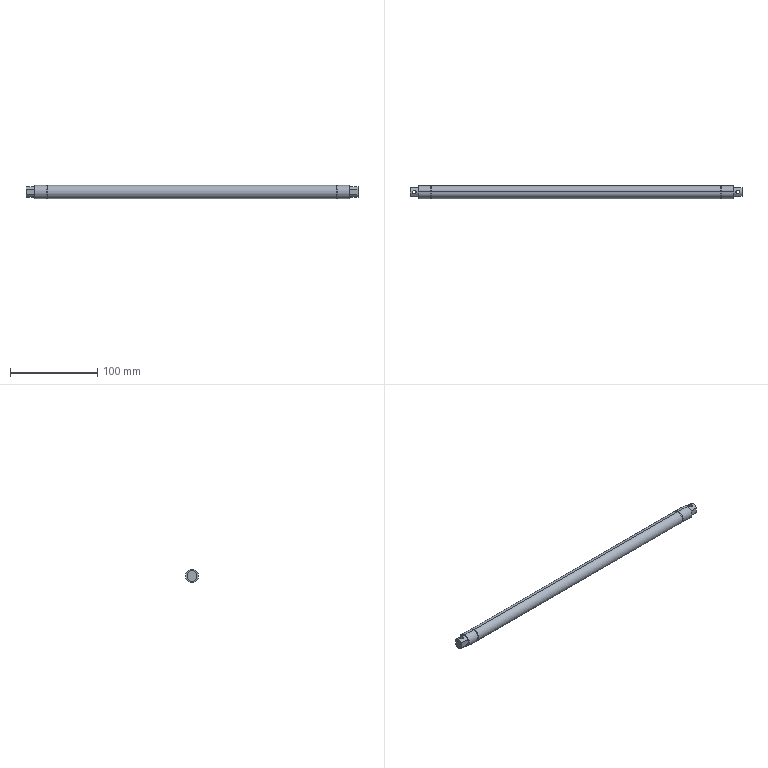Component | SolidWorks | 01-12MarkingMachinePrintingRollerAxis-1 | 1 solid | 32 faces | box 380 x 15 x 15 mm | volume 65336 mm3 | cylinder 20 | plane 12 | commonest cylinder face diameters 15 x6 12 x6 4.2 x4 14.3 x4 | material A3 Steel
build123d program:
from build123d import *

# Parameters (mm, degrees)
SKETCH2_W          = 10
SKETCH2_H          = 1
CUT_EXTRUDE1_DEPTH = 191.296
M5_TAPPED_HOLE1_D  = 4.2


with BuildPart() as part:
    # Sketch1 → Revolve1 (revolve)
    with BuildSketch(Plane.XY, mode=Mode.PRIVATE) as revolve1_sk:
        Polygon((-190, 0), (-190, 6), (-180, 6), (-180, 7.5), (-166.1, 7.5), (-166.1, 7.15), (-165, 7.15), (-165, 7.5), (165, 7.5), (165, 7.15), (166.1, 7.15), (166.1, 7.5), (180, 7.5), (180, 6), (190, 6), (190, 0), align=None)
    revolve(revolve1_sk.sketch.rotate(Axis((-253.202, 0, 0), (1, 0, 0)), 90), axis=Axis((-253.202, 0, 0), (1, 0, 0)))

    # Sketch2 → Cut-Extrude1 (cut, symmetric)
    with BuildSketch(Plane.XY):
        with Locations((-185, 5.5)):
            Rectangle(SKETCH2_W, SKETCH2_H)
        with Locations((-185, -5.5)):
            Rectangle(SKETCH2_W, SKETCH2_H)
    cut_extrude1 = extrude(amount=CUT_EXTRUDE1_DEPTH, both=True, mode=Mode.SUBTRACT)

    # M5 Tapped Hole1 (through all)
    with Locations(Plane(origin=(-185, 0, 6), x_dir=(0, 1, 0), z_dir=(0, 0, 1))):
        with Locations((0, 0)):
            m5_tapped_hole1 = Hole(M5_TAPPED_HOLE1_D / 2)

    # Mirror1: Cut-Extrude1, M5 Tapped Hole1 across plane
    add(cut_extrude1.mirror(Plane(origin=(0, 0, 0), x_dir=(0, 0, 1), z_dir=(1, 0, 0))), mode=Mode.SUBTRACT)
    add(m5_tapped_hole1.mirror(Plane(origin=(0, 0, 0), x_dir=(0, 0, 1), z_dir=(1, 0, 0))), mode=Mode.SUBTRACT)


solid = part.part

# Placed as in the assembly
solid = solid.moved(Location((-256.91, 2.41, 6.568), (0, 0, 0)))